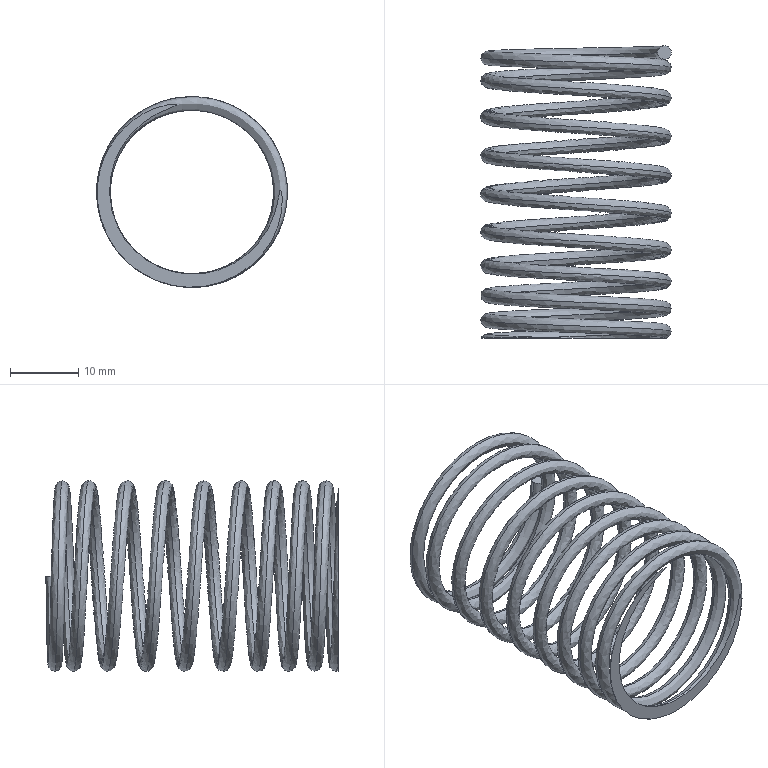Component | SolidWorks | spring2-1 | 1 solid | 4 faces | volume 2452 mm3 | spline 2 | plane 2